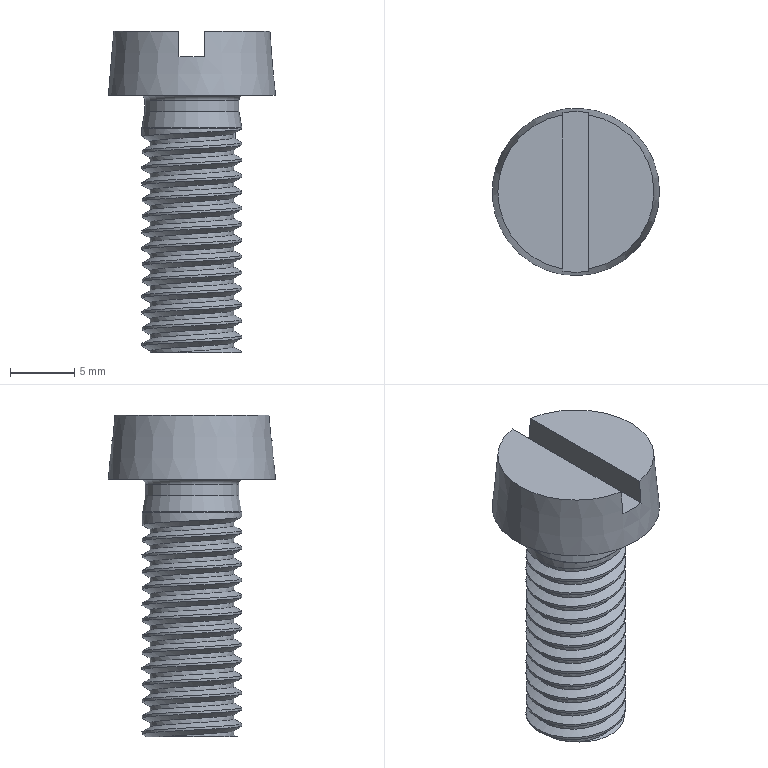Component | NX | M8_SLOTTED_BOLT_2 | 1 solid | 19 faces | volume 1466 mm3 | plane 10 | cylinder 4 | cone 2 | spline 2 | torus 1 | commonest cylinder face diameters 7.309 x1 6.619 x1 7.76 x1 6.51 x1